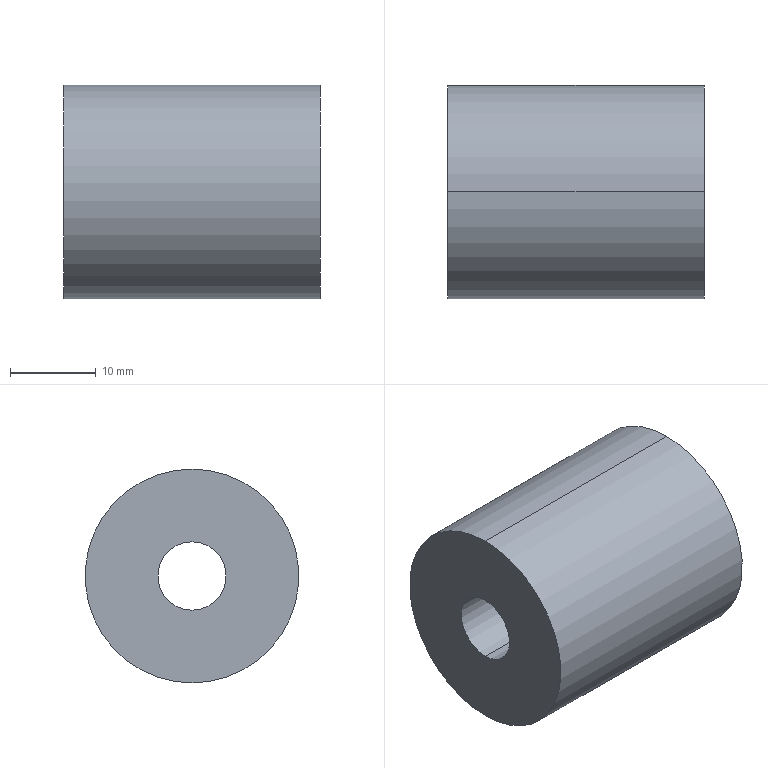Component | SolidWorks | 8X8X30Coupling-1 | 1 solid | 6 faces | box 30 x 25 x 25 mm | volume 13218 mm3 | cylinder 4 | plane 2 | commonest cylinder face diameters 8 x2 25 x2 | material AISI 1045 Steel, Cold Drawn
build123d program:
from build123d import *

# Parameters (mm, degrees)
SKETCH1_R           = 12.5
SKETCH1_R_2         = 4
BOSS_EXTRUDE1_DEPTH = 30


with BuildPart() as part:
    # Sketch1 → Boss-Extrude1 (new body)
    with BuildSketch(Plane(origin=(0, 0, 0), x_dir=(1, 0, 0), z_dir=(0, 1, 0))):
        with Locations(Location((0, 0, 0), (0, 0, 270))):
            Circle(SKETCH1_R)
        with Locations(Location((0, 0, 0), (0, 0, 270))):
            Circle(SKETCH1_R_2, mode=Mode.SUBTRACT)
    extrude(amount=BOSS_EXTRUDE1_DEPTH)


solid = part.part

# Placed as in the assembly
solid = solid.moved(Location((130.062, 15.116, 349), (0, 0, 90)))
STEP:
#1=COLOUR_RGB('',0.7922,0.8196,0.9333);
#2=FILL_AREA_STYLE_COLOUR('',#1);
#3=FILL_AREA_STYLE('',(#2));
#4=SURFACE_STYLE_FILL_AREA(#3);
#5=SURFACE_SIDE_STYLE('',(#4));
#6=SURFACE_STYLE_USAGE(.BOTH.,#5);
#7=PRESENTATION_STYLE_ASSIGNMENT((#6));
#8=CARTESIAN_POINT('',(3.939,0.5951,13.583));
#9=VERTEX_POINT('',#8);
#10=CARTESIAN_POINT('',(3.939,0.5951,13.898));
#11=VERTEX_POINT('',#10);
#12=CARTESIAN_POINT('',(3.939,0.5951,13.74));
#13=DIRECTION('',(-1.,0.,0.));
#14=DIRECTION('',(0.,0.,1.));
#15=AXIS2_PLACEMENT_3D('',#12,#13,#14);
#16=CIRCLE('',#15,0.1575);
#17=EDGE_CURVE('',#9,#11,#16,.T.);
#18=ORIENTED_EDGE('',*,*,#17,.T.);
#19=CARTESIAN_POINT('',(5.121,0.5951,13.898));
#20=VERTEX_POINT('',#19);
#21=CARTESIAN_POINT('',(3.939,0.5951,13.898));
#22=DIRECTION('',(1.,0.,0.));
#23=VECTOR('',#22,39.37);
#24=LINE('',#21,#23);
#25=EDGE_CURVE('',#11,#20,#24,.T.);
#26=ORIENTED_EDGE('',*,*,#25,.T.);
#27=CARTESIAN_POINT('',(5.121,0.5951,13.583));
#28=VERTEX_POINT('',#27);
#29=CARTESIAN_POINT('',(5.121,0.5951,13.74));
#30=DIRECTION('',(-1.,0.,0.));
#31=DIRECTION('',(0.,0.,1.));
#32=AXIS2_PLACEMENT_3D('',#29,#30,#31);
#33=CIRCLE('',#32,0.1575);
#34=EDGE_CURVE('',#28,#20,#33,.T.);
#35=ORIENTED_EDGE('',*,*,#34,.F.);
#36=CARTESIAN_POINT('',(3.939,0.5951,13.583));
#37=DIRECTION('',(1.,0.,0.));
#38=VECTOR('',#37,39.37);
#39=LINE('',#36,#38);
#40=EDGE_CURVE('',#9,#28,#39,.T.);
#41=ORIENTED_EDGE('',*,*,#40,.F.);
#42=EDGE_LOOP('',(#18,#26,#35,#41));
#43=FACE_OUTER_BOUND('',#42,.T.);
#44=CARTESIAN_POINT('',(3.939,0.5951,13.74));
#45=DIRECTION('',(1.,0.,0.));
#46=DIRECTION('',(0.,0.,-1.));
#47=AXIS2_PLACEMENT_3D('',#44,#45,#46);
#48=CYLINDRICAL_SURFACE('',#47,0.1575);
#49=ADVANCED_FACE('',(#43),#48,.F.);
#50=CARTESIAN_POINT('',(3.939,0.5951,14.232));
#51=VERTEX_POINT('',#50);
#52=CARTESIAN_POINT('',(3.939,0.5951,13.248));
#53=VERTEX_POINT('',#52);
#54=CARTESIAN_POINT('',(3.939,0.5951,13.74));
#55=DIRECTION('',(-1.,0.,0.));
#56=DIRECTION('',(0.,0.,1.));
#57=AXIS2_PLACEMENT_3D('',#54,#55,#56);
#58=CIRCLE('',#57,0.4921);
#59=EDGE_CURVE('',#51,#53,#58,.T.);
#60=ORIENTED_EDGE('',*,*,#59,.F.);
#61=CARTESIAN_POINT('',(5.121,0.5951,14.232));
#62=VERTEX_POINT('',#61);
#63=CARTESIAN_POINT('',(3.939,0.5951,14.232));
#64=DIRECTION('',(1.,0.,0.));
#65=VECTOR('',#64,39.37);
#66=LINE('',#63,#65);
#67=EDGE_CURVE('',#51,#62,#66,.T.);
#68=ORIENTED_EDGE('',*,*,#67,.T.);
#69=CARTESIAN_POINT('',(5.121,0.5951,13.248));
#70=VERTEX_POINT('',#69);
#71=CARTESIAN_POINT('',(5.121,0.5951,13.74));
#72=DIRECTION('',(-1.,0.,0.));
#73=DIRECTION('',(0.,0.,1.));
#74=AXIS2_PLACEMENT_3D('',#71,#72,#73);
#75=CIRCLE('',#74,0.4921);
#76=EDGE_CURVE('',#62,#70,#75,.T.);
#77=ORIENTED_EDGE('',*,*,#76,.T.);
#78=CARTESIAN_POINT('',(3.939,0.5951,13.248));
#79=DIRECTION('',(1.,0.,0.));
#80=VECTOR('',#79,39.37);
#81=LINE('',#78,#80);
#82=EDGE_CURVE('',#53,#70,#81,.T.);
#83=ORIENTED_EDGE('',*,*,#82,.F.);
#84=EDGE_LOOP('',(#60,#68,#77,#83));
#85=FACE_OUTER_BOUND('',#84,.T.);
#86=CARTESIAN_POINT('',(3.939,0.5951,13.74));
#87=DIRECTION('',(1.,0.,0.));
#88=DIRECTION('',(0.,0.,-1.));
#89=AXIS2_PLACEMENT_3D('',#86,#87,#88);
#90=CYLINDRICAL_SURFACE('',#89,0.4921);
#91=ADVANCED_FACE('',(#85),#90,.T.);
#92=CARTESIAN_POINT('',(3.939,0.5951,13.74));
#93=DIRECTION('',(-1.,0.,0.));
#94=DIRECTION('',(0.,0.,1.));
#95=AXIS2_PLACEMENT_3D('',#92,#93,#94);
#96=CIRCLE('',#95,0.4921);
#97=EDGE_CURVE('',#53,#51,#96,.T.);
#98=ORIENTED_EDGE('',*,*,#97,.T.);
#99=ORIENTED_EDGE('',*,*,#59,.T.);
#100=EDGE_LOOP('',(#98,#99));
#101=FACE_OUTER_BOUND('',#100,.T.);
#102=ORIENTED_EDGE('',*,*,#17,.F.);
#103=CARTESIAN_POINT('',(3.939,0.5951,13.74));
#104=DIRECTION('',(-1.,0.,0.));
#105=DIRECTION('',(0.,0.,1.));
#106=AXIS2_PLACEMENT_3D('',#103,#104,#105);
#107=CIRCLE('',#106,0.1575);
#108=EDGE_CURVE('',#11,#9,#107,.T.);
#109=ORIENTED_EDGE('',*,*,#108,.F.);
#110=EDGE_LOOP('',(#102,#109));
#111=FACE_BOUND('',#110,.T.);
#112=CARTESIAN_POINT('',(3.939,0.5951,13.74));
#113=DIRECTION('',(-1.,0.,0.));
#114=DIRECTION('',(0.,0.,1.));
#115=AXIS2_PLACEMENT_3D('',#112,#113,#114);
#116=PLANE('',#115);
#117=ADVANCED_FACE('',(#101,#111),#116,.T.);
#118=CARTESIAN_POINT('',(5.121,0.5951,13.74));
#119=DIRECTION('',(-1.,0.,0.));
#120=DIRECTION('',(0.,0.,1.));
#121=AXIS2_PLACEMENT_3D('',#118,#119,#120);
#122=CIRCLE('',#121,0.4921);
#123=EDGE_CURVE('',#70,#62,#122,.T.);
#124=ORIENTED_EDGE('',*,*,#123,.F.);
#125=ORIENTED_EDGE('',*,*,#76,.F.);
#126=EDGE_LOOP('',(#124,#125));
#127=FACE_OUTER_BOUND('',#126,.T.);
#128=ORIENTED_EDGE('',*,*,#34,.T.);
#129=CARTESIAN_POINT('',(5.121,0.5951,13.74));
#130=DIRECTION('',(-1.,0.,0.));
#131=DIRECTION('',(0.,0.,1.));
#132=AXIS2_PLACEMENT_3D('',#129,#130,#131);
#133=CIRCLE('',#132,0.1575);
#134=EDGE_CURVE('',#20,#28,#133,.T.);
#135=ORIENTED_EDGE('',*,*,#134,.T.);
#136=EDGE_LOOP('',(#128,#135));
#137=FACE_BOUND('',#136,.T.);
#138=CARTESIAN_POINT('',(5.121,0.5951,13.74));
#139=DIRECTION('',(-1.,0.,0.));
#140=DIRECTION('',(0.,0.,1.));
#141=AXIS2_PLACEMENT_3D('',#138,#139,#140);
#142=PLANE('',#141);
#143=ADVANCED_FACE('',(#127,#137),#142,.F.);
#144=ORIENTED_EDGE('',*,*,#67,.F.);
#145=ORIENTED_EDGE('',*,*,#97,.F.);
#146=ORIENTED_EDGE('',*,*,#82,.T.);
#147=ORIENTED_EDGE('',*,*,#123,.T.);
#148=EDGE_LOOP('',(#144,#145,#146,#147));
#149=FACE_OUTER_BOUND('',#148,.T.);
#150=CARTESIAN_POINT('',(3.939,0.5951,13.74));
#151=DIRECTION('',(1.,0.,0.));
#152=DIRECTION('',(0.,0.,-1.));
#153=AXIS2_PLACEMENT_3D('',#150,#151,#152);
#154=CYLINDRICAL_SURFACE('',#153,0.4921);
#155=ADVANCED_FACE('',(#149),#154,.T.);
#156=ORIENTED_EDGE('',*,*,#25,.F.);
#157=ORIENTED_EDGE('',*,*,#108,.T.);
#158=ORIENTED_EDGE('',*,*,#40,.T.);
#159=ORIENTED_EDGE('',*,*,#134,.F.);
#160=EDGE_LOOP('',(#156,#157,#158,#159));
#161=FACE_OUTER_BOUND('',#160,.T.);
#162=CARTESIAN_POINT('',(3.939,0.5951,13.74));
#163=DIRECTION('',(1.,0.,0.));
#164=DIRECTION('',(0.,0.,-1.));
#165=AXIS2_PLACEMENT_3D('',#162,#163,#164);
#166=CYLINDRICAL_SURFACE('',#165,0.1575);
#167=ADVANCED_FACE('',(#161),#166,.F.);
#168=CLOSED_SHELL('',(#49,#91,#117,#143,#155,#167));
#169=MANIFOLD_SOLID_BREP('',#168);
#170=STYLED_ITEM('',(#7),#169);
#171=PRESENTATION_LAYER_ASSIGNMENT('','',(#170));
#172=(LENGTH_UNIT()NAMED_UNIT(*)SI_UNIT($,.METRE.));
#173=LENGTH_MEASURE_WITH_UNIT(LENGTH_MEASURE(0.0254),#172);
#174=DIMENSIONAL_EXPONENTS(1.,0.,0.,0.,0.,0.,0.);
#175=(CONVERSION_BASED_UNIT('',#173)LENGTH_UNIT()NAMED_UNIT(#174));
#176=UNCERTAINTY_MEASURE_WITH_UNIT(LENGTH_MEASURE(0.00001),#175,'','');
#177=(NAMED_UNIT(*)PLANE_ANGLE_UNIT()SI_UNIT($,.RADIAN.));
#178=(NAMED_UNIT(*)SI_UNIT($,.STERADIAN.)SOLID_ANGLE_UNIT());
#179=(GEOMETRIC_REPRESENTATION_CONTEXT(3)GLOBAL_UNCERTAINTY_ASSIGNED_CONTEXT((#176))GLOBAL_UNIT_ASSIGNED_CONTEXT((#175,#177,#178))REPRESENTATION_CONTEXT('',''));
#180=MECHANICAL_DESIGN_GEOMETRIC_PRESENTATION_REPRESENTATION('',(#170),#179);
#181=CARTESIAN_POINT('',(0.,0.,0.));
#182=DIRECTION('',(0.,0.,1.));
#183=DIRECTION('',(1.,0.,0.));
#184=AXIS2_PLACEMENT_3D('',#181,#182,#183);
#185=(LENGTH_UNIT()NAMED_UNIT(*)SI_UNIT($,.METRE.));
#186=LENGTH_MEASURE_WITH_UNIT(LENGTH_MEASURE(0.0254),#185);
#187=DIMENSIONAL_EXPONENTS(1.,0.,0.,0.,0.,0.,0.);
#188=(CONVERSION_BASED_UNIT('',#186)LENGTH_UNIT()NAMED_UNIT(#187));
#189=UNCERTAINTY_MEASURE_WITH_UNIT(LENGTH_MEASURE(0.00001),#188,'','');
#190=(NAMED_UNIT(*)PLANE_ANGLE_UNIT()SI_UNIT($,.RADIAN.));
#191=(NAMED_UNIT(*)SI_UNIT($,.STERADIAN.)SOLID_ANGLE_UNIT());
#192=(GEOMETRIC_REPRESENTATION_CONTEXT(3)GLOBAL_UNCERTAINTY_ASSIGNED_CONTEXT((#189))GLOBAL_UNIT_ASSIGNED_CONTEXT((#188,#190,#191))REPRESENTATION_CONTEXT('',''));
#193=ADVANCED_BREP_SHAPE_REPRESENTATION('',(#169,#184),#192);